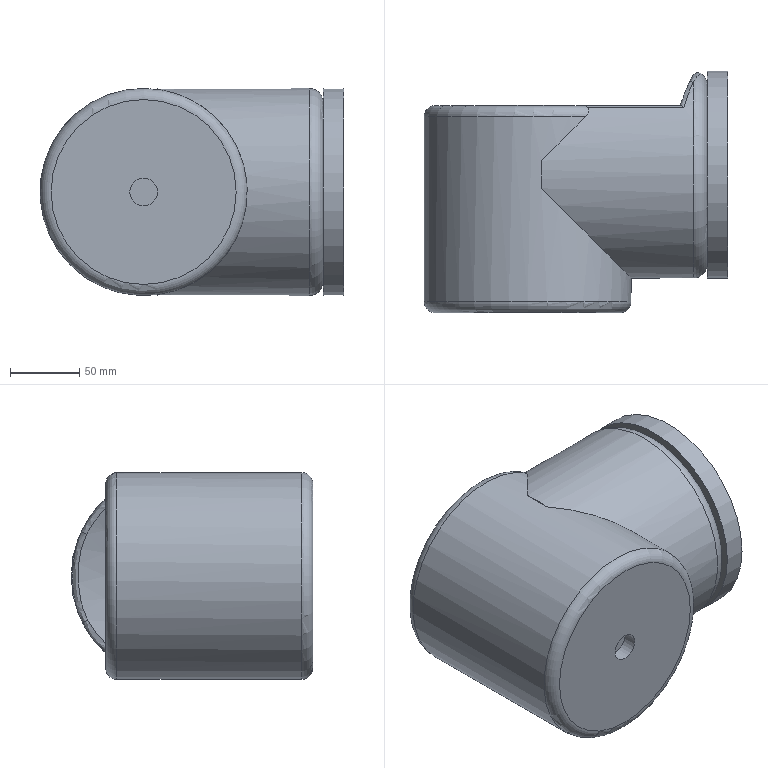Component | NX | 6_WRIST | 2 solids | 26 faces | box 220 x 175 x 150 mm | volume 3966600 mm3 | cylinder 10 | plane 10 | torus 3 | spline 3 | commonest cylinder face diameters 150 x4 20 x3 10 x2 300 x1
STEP:
#1=CARTESIAN_POINT('',(0.,0.,0.));
#2=DIRECTION('',(0.,0.,1.));
#3=DIRECTION('',(1.,0.,0.));
#4=AXIS2_PLACEMENT_3D('',#1,#2,#3);
#5=(LENGTH_UNIT()NAMED_UNIT(*)SI_UNIT(.MILLI.,.METRE.));
#6=UNCERTAINTY_MEASURE_WITH_UNIT(LENGTH_MEASURE(0.0508),#5,'','');
#7=(NAMED_UNIT(*)PLANE_ANGLE_UNIT()SI_UNIT($,.RADIAN.));
#8=PLANE_ANGLE_MEASURE_WITH_UNIT(PLANE_ANGLE_MEASURE(0.01745),#7);
#9=DIMENSIONAL_EXPONENTS(0.,0.,0.,0.,0.,0.,0.);
#10=(CONVERSION_BASED_UNIT('',#8)NAMED_UNIT(#9)PLANE_ANGLE_UNIT());
#11=(NAMED_UNIT(*)SI_UNIT($,.STERADIAN.)SOLID_ANGLE_UNIT());
#12=(GEOMETRIC_REPRESENTATION_CONTEXT(3)GLOBAL_UNCERTAINTY_ASSIGNED_CONTEXT((#6))GLOBAL_UNIT_ASSIGNED_CONTEXT((#5,#10,#11))REPRESENTATION_CONTEXT('',''));
#13=SHAPE_REPRESENTATION('',(#4),#12);
#14=CARTESIAN_POINT('',(0.,0.,-237.5));
#15=DIRECTION('',(0.,0.,1.));
#16=DIRECTION('',(1.,0.,0.));
#17=AXIS2_PLACEMENT_3D('',#14,#15,#16);
#18=CONSTRUCTIVE_GEOMETRY_REPRESENTATION('',(#17),#12);
#19=CONSTRUCTIVE_GEOMETRY_REPRESENTATION_RELATIONSHIP('','',#13,#18);
#20=VALUE_REPRESENTATION_ITEM('',COUNT_MEASURE(0.));
#21=REPRESENTATION('',(#20),#12);
#22=VALUE_REPRESENTATION_ITEM('',COUNT_MEASURE(0.));
#23=REPRESENTATION('',(#22),#12);
#24=CARTESIAN_POINT('',(1171.262,-87.,1644.589));
#25=VERTEX_POINT('',#24);
#26=CARTESIAN_POINT('',(1171.262,-87.,1569.589));
#27=DIRECTION('',(0.,1.,0.));
#28=DIRECTION('',(0.,0.,1.));
#29=AXIS2_PLACEMENT_3D('',#26,#27,#28);
#30=CIRCLE('',#29,75.);
#31=EDGE_CURVE('',#25,#25,#30,.T.);
#32=ORIENTED_EDGE('',*,*,#31,.T.);
#33=EDGE_LOOP('',(#32));
#34=FACE_BOUND('',#33,.T.);
#35=CARTESIAN_POINT('',(1181.262,15.,1495.259));
#36=VERTEX_POINT('',#35);
#37=CARTESIAN_POINT('',(1213.262,47.,1507.452));
#38=VERTEX_POINT('',#37);
#39=CARTESIAN_POINT('',(1171.262,5.,1569.589));
#40=DIRECTION('',(0.7071,-0.7071,0.));
#41=DIRECTION('',(0.7071,0.7071,0.));
#42=AXIS2_PLACEMENT_3D('',#39,#40,#41);
#43=ELLIPSE('',#42,106.066,75.);
#44=EDGE_CURVE('',#36,#38,#43,.T.);
#45=ORIENTED_EDGE('',*,*,#44,.F.);
#46=CARTESIAN_POINT('',(1181.262,-5.,1495.259));
#47=VERTEX_POINT('',#46);
#48=CARTESIAN_POINT('',(1181.262,-95.,1495.259));
#49=DIRECTION('',(0.,1.,0.));
#50=VECTOR('',#49,1.);
#51=LINE('',#48,#50);
#52=EDGE_CURVE('',#47,#36,#51,.T.);
#53=ORIENTED_EDGE('',*,*,#52,.F.);
#54=CARTESIAN_POINT('',(1181.262,-5.,1643.92));
#55=VERTEX_POINT('',#54);
#56=CARTESIAN_POINT('',(1171.262,5.,1569.589));
#57=DIRECTION('',(0.7071,0.7071,0.));
#58=DIRECTION('',(-0.7071,0.7071,0.));
#59=AXIS2_PLACEMENT_3D('',#56,#57,#58);
#60=ELLIPSE('',#59,106.066,75.);
#61=EDGE_CURVE('',#55,#47,#60,.T.);
#62=ORIENTED_EDGE('',*,*,#61,.F.);
#63=CARTESIAN_POINT('',(1181.262,15.,1643.92));
#64=VERTEX_POINT('',#63);
#65=CARTESIAN_POINT('',(1181.262,-95.,1643.92));
#66=DIRECTION('',(0.,-1.,0.));
#67=VECTOR('',#66,1.);
#68=LINE('',#65,#67);
#69=EDGE_CURVE('',#64,#55,#68,.T.);
#70=ORIENTED_EDGE('',*,*,#69,.F.);
#71=CARTESIAN_POINT('',(1213.262,47.,1631.726));
#72=VERTEX_POINT('',#71);
#73=CARTESIAN_POINT('',(1171.262,5.,1569.589));
#74=DIRECTION('',(0.7071,-0.7071,0.));
#75=DIRECTION('',(0.7071,0.7071,0.));
#76=AXIS2_PLACEMENT_3D('',#73,#74,#75);
#77=ELLIPSE('',#76,106.066,75.);
#78=EDGE_CURVE('',#72,#64,#77,.T.);
#79=ORIENTED_EDGE('',*,*,#78,.F.);
#80=CARTESIAN_POINT('',(1171.262,47.,1569.589));
#81=DIRECTION('',(0.,-1.,0.));
#82=DIRECTION('',(0.,0.,1.));
#83=AXIS2_PLACEMENT_3D('',#80,#81,#82);
#84=CIRCLE('',#83,75.);
#85=EDGE_CURVE('',#72,#38,#84,.T.);
#86=ORIENTED_EDGE('',*,*,#85,.T.);
#87=EDGE_LOOP('',(#45,#53,#62,#70,#79,#86));
#88=FACE_BOUND('',#87,.T.);
#89=CARTESIAN_POINT('',(1171.262,-95.,1569.589));
#90=DIRECTION('',(0.,1.,0.));
#91=DIRECTION('',(0.,0.,-1.));
#92=AXIS2_PLACEMENT_3D('',#89,#90,#91);
#93=CYLINDRICAL_SURFACE('',#92,75.);
#94=ADVANCED_FACE('',(#34,#88),#93,.T.);
#95=CARTESIAN_POINT('',(1214.726,53.214,1512.14));
#96=VERTEX_POINT('',#95);
#97=CARTESIAN_POINT('',(1211.436,55.,1515.97));
#98=VERTEX_POINT('',#97);
#99=CARTESIAN_POINT('',(1214.726,53.214,1512.14));
#100=CARTESIAN_POINT('',(1213.654,54.361,1513.102));
#101=CARTESIAN_POINT('',(1212.548,55.,1514.535));
#102=CARTESIAN_POINT('',(1211.436,55.,1515.97));
#103=B_SPLINE_CURVE_WITH_KNOTS('',3,(#99,#100,#101,#102),.UNSPECIFIED.,.F.,.F.,(4,4),(0.,1.),.UNSPECIFIED.);
#104=EDGE_CURVE('',#96,#98,#103,.T.);
#105=ORIENTED_EDGE('',*,*,#104,.F.);
#106=CARTESIAN_POINT('',(1214.726,53.214,1512.14));
#107=CARTESIAN_POINT('',(1215.561,52.321,1511.39));
#108=CARTESIAN_POINT('',(1215.653,51.105,1510.418));
#109=CARTESIAN_POINT('',(1214.918,48.916,1508.776));
#110=CARTESIAN_POINT('',(1214.17,47.908,1508.066));
#111=CARTESIAN_POINT('',(1213.262,47.,1507.452));
#112=B_SPLINE_CURVE_WITH_KNOTS('',3,(#106,#107,#108,#109,#110,#111),.UNSPECIFIED.,.F.,.F.,(4,2,4),(0.,0.5,1.),.UNSPECIFIED.);
#113=EDGE_CURVE('',#96,#38,#112,.T.);
#114=ORIENTED_EDGE('',*,*,#113,.T.);
#115=ORIENTED_EDGE('',*,*,#85,.F.);
#116=CARTESIAN_POINT('',(1214.726,53.214,1627.038));
#117=VERTEX_POINT('',#116);
#118=CARTESIAN_POINT('',(1213.262,47.,1631.726));
#119=CARTESIAN_POINT('',(1214.171,47.909,1631.112));
#120=CARTESIAN_POINT('',(1214.92,48.919,1630.4));
#121=CARTESIAN_POINT('',(1215.654,51.11,1628.756));
#122=CARTESIAN_POINT('',(1215.562,52.32,1627.789));
#123=CARTESIAN_POINT('',(1214.726,53.214,1627.038));
#124=B_SPLINE_CURVE_WITH_KNOTS('',3,(#118,#119,#120,#121,#122,#123),.UNSPECIFIED.,.F.,.F.,(4,2,4),(0.,0.5,1.),.UNSPECIFIED.);
#125=EDGE_CURVE('',#72,#117,#124,.T.);
#126=ORIENTED_EDGE('',*,*,#125,.T.);
#127=CARTESIAN_POINT('',(1211.436,55.,1623.208));
#128=VERTEX_POINT('',#127);
#129=CARTESIAN_POINT('',(1211.436,55.,1623.208));
#130=CARTESIAN_POINT('',(1212.549,55.,1624.644));
#131=CARTESIAN_POINT('',(1213.654,54.361,1626.076));
#132=CARTESIAN_POINT('',(1214.726,53.214,1627.038));
#133=B_SPLINE_CURVE_WITH_KNOTS('',3,(#129,#130,#131,#132),.UNSPECIFIED.,.F.,.F.,(4,4),(0.,1.),.UNSPECIFIED.);
#134=EDGE_CURVE('',#128,#117,#133,.T.);
#135=ORIENTED_EDGE('',*,*,#134,.F.);
#136=CARTESIAN_POINT('',(1171.262,55.,1569.589));
#137=DIRECTION('',(0.,1.,0.));
#138=DIRECTION('',(0.,0.,1.));
#139=AXIS2_PLACEMENT_3D('',#136,#137,#138);
#140=CIRCLE('',#139,67.);
#141=EDGE_CURVE('',#98,#128,#140,.T.);
#142=ORIENTED_EDGE('',*,*,#141,.F.);
#143=EDGE_LOOP('',(#105,#114,#115,#126,#135,#142));
#144=FACE_OUTER_BOUND('',#143,.T.);
#145=CARTESIAN_POINT('',(1171.262,47.,1569.589));
#146=DIRECTION('',(0.,-1.,0.));
#147=DIRECTION('',(0.,0.,1.));
#148=AXIS2_PLACEMENT_3D('',#145,#146,#147);
#149=TOROIDAL_SURFACE('',#148,67.,8.);
#150=ADVANCED_FACE('',(#144),#149,.T.);
#151=CARTESIAN_POINT('',(1171.262,-95.,1636.589));
#152=VERTEX_POINT('',#151);
#153=CARTESIAN_POINT('',(1171.262,-95.,1569.589));
#154=DIRECTION('',(0.,-1.,0.));
#155=DIRECTION('',(0.,0.,1.));
#156=AXIS2_PLACEMENT_3D('',#153,#154,#155);
#157=CIRCLE('',#156,67.);
#158=EDGE_CURVE('',#152,#152,#157,.T.);
#159=ORIENTED_EDGE('',*,*,#158,.T.);
#160=EDGE_LOOP('',(#159));
#161=FACE_BOUND('',#160,.T.);
#162=CARTESIAN_POINT('',(1161.262,-95.,1569.589));
#163=VERTEX_POINT('',#162);
#164=CARTESIAN_POINT('',(1171.262,-95.,1569.589));
#165=DIRECTION('',(0.,1.,0.));
#166=DIRECTION('',(-1.,0.,0.));
#167=AXIS2_PLACEMENT_3D('',#164,#165,#166);
#168=CIRCLE('',#167,10.);
#169=EDGE_CURVE('',#163,#163,#168,.T.);
#170=ORIENTED_EDGE('',*,*,#169,.T.);
#171=EDGE_LOOP('',(#170));
#172=FACE_BOUND('',#171,.T.);
#173=CARTESIAN_POINT('',(1171.262,-95.,1569.589));
#174=DIRECTION('',(0.,-1.,0.));
#175=DIRECTION('',(0.,0.,1.));
#176=AXIS2_PLACEMENT_3D('',#173,#174,#175);
#177=PLANE('',#176);
#178=ADVANCED_FACE('',(#161,#172),#177,.T.);
#179=ORIENTED_EDGE('',*,*,#141,.T.);
#180=CARTESIAN_POINT('',(1281.893,55.,1623.208));
#181=VERTEX_POINT('',#180);
#182=CARTESIAN_POINT('',(1279.425,55.,1623.208));
#183=DIRECTION('',(1.,0.,0.));
#184=VECTOR('',#183,1.);
#185=LINE('',#182,#184);
#186=EDGE_CURVE('',#128,#181,#185,.T.);
#187=ORIENTED_EDGE('',*,*,#186,.T.);
#188=CARTESIAN_POINT('',(1282.026,55.,1618.665));
#189=VERTEX_POINT('',#188);
#190=CARTESIAN_POINT('',(1281.893,55.,1623.208));
#191=CARTESIAN_POINT('',(1281.349,55.,1621.739));
#192=CARTESIAN_POINT('',(1281.508,55.,1620.133));
#193=CARTESIAN_POINT('',(1282.026,55.,1618.665));
#194=B_SPLINE_CURVE_WITH_KNOTS('',3,(#190,#191,#192,#193),.UNSPECIFIED.,.F.,.F.,(4,4),(0.,1.),.UNSPECIFIED.);
#195=EDGE_CURVE('',#181,#189,#194,.T.);
#196=ORIENTED_EDGE('',*,*,#195,.T.);
#197=CARTESIAN_POINT('',(1282.635,55.,1520.467));
#198=VERTEX_POINT('',#197);
#199=CARTESIAN_POINT('',(1140.597,55.,1568.688));
#200=DIRECTION('',(0.,1.,0.));
#201=DIRECTION('',(1.,0.,0.));
#202=AXIS2_PLACEMENT_3D('',#199,#200,#201);
#203=CIRCLE('',#202,150.);
#204=EDGE_CURVE('',#189,#198,#203,.T.);
#205=ORIENTED_EDGE('',*,*,#204,.T.);
#206=CARTESIAN_POINT('',(1282.546,55.,1515.97));
#207=VERTEX_POINT('',#206);
#208=CARTESIAN_POINT('',(1282.635,55.,1520.467));
#209=CARTESIAN_POINT('',(1282.14,55.,1519.009));
#210=CARTESIAN_POINT('',(1282.002,55.,1517.42));
#211=CARTESIAN_POINT('',(1282.546,55.,1515.97));
#212=B_SPLINE_CURVE_WITH_KNOTS('',3,(#208,#209,#210,#211),.UNSPECIFIED.,.F.,.F.,(4,4),(0.,1.),.UNSPECIFIED.);
#213=EDGE_CURVE('',#198,#207,#212,.T.);
#214=ORIENTED_EDGE('',*,*,#213,.T.);
#215=CARTESIAN_POINT('',(1181.262,55.,1515.97));
#216=DIRECTION('',(-1.,0.,0.));
#217=VECTOR('',#216,1.);
#218=LINE('',#215,#217);
#219=EDGE_CURVE('',#207,#98,#218,.T.);
#220=ORIENTED_EDGE('',*,*,#219,.T.);
#221=EDGE_LOOP('',(#179,#187,#196,#205,#214,#220));
#222=FACE_BOUND('',#221,.T.);
#223=CARTESIAN_POINT('',(1171.262,55.,1579.589));
#224=VERTEX_POINT('',#223);
#225=CARTESIAN_POINT('',(1171.262,55.,1569.589));
#226=DIRECTION('',(0.,-1.,0.));
#227=DIRECTION('',(0.,0.,1.));
#228=AXIS2_PLACEMENT_3D('',#225,#226,#227);
#229=CIRCLE('',#228,10.);
#230=EDGE_CURVE('',#224,#224,#229,.T.);
#231=ORIENTED_EDGE('',*,*,#230,.T.);
#232=EDGE_LOOP('',(#231));
#233=FACE_BOUND('',#232,.T.);
#234=CARTESIAN_POINT('',(1171.262,55.,1569.589));
#235=DIRECTION('',(0.,-1.,0.));
#236=DIRECTION('',(0.,0.,1.));
#237=AXIS2_PLACEMENT_3D('',#234,#235,#236);
#238=PLANE('',#237);
#239=ADVANCED_FACE('',(#222,#233),#238,.F.);
#240=ORIENTED_EDGE('',*,*,#230,.F.);
#241=EDGE_LOOP('',(#240));
#242=FACE_BOUND('',#241,.T.);
#243=CARTESIAN_POINT('',(1171.262,45.,1579.589));
#244=VERTEX_POINT('',#243);
#245=CARTESIAN_POINT('',(1171.262,45.,1569.589));
#246=DIRECTION('',(0.,-1.,0.));
#247=DIRECTION('',(0.,0.,1.));
#248=AXIS2_PLACEMENT_3D('',#245,#246,#247);
#249=CIRCLE('',#248,10.);
#250=EDGE_CURVE('',#244,#244,#249,.T.);
#251=ORIENTED_EDGE('',*,*,#250,.T.);
#252=EDGE_LOOP('',(#251));
#253=FACE_BOUND('',#252,.T.);
#254=CARTESIAN_POINT('',(1171.262,55.,1569.589));
#255=DIRECTION('',(0.,-1.,0.));
#256=DIRECTION('',(0.,0.,1.));
#257=AXIS2_PLACEMENT_3D('',#254,#255,#256);
#258=CYLINDRICAL_SURFACE('',#257,10.);
#259=ADVANCED_FACE('',(#242,#253),#258,.F.);
#260=ORIENTED_EDGE('',*,*,#250,.F.);
#261=EDGE_LOOP('',(#260));
#262=FACE_OUTER_BOUND('',#261,.T.);
#263=CARTESIAN_POINT('',(1171.262,45.,1569.589));
#264=DIRECTION('',(0.,-1.,0.));
#265=DIRECTION('',(0.,0.,1.));
#266=AXIS2_PLACEMENT_3D('',#263,#264,#265);
#267=PLANE('',#266);
#268=ADVANCED_FACE('',(#262),#267,.F.);
#269=ORIENTED_EDGE('',*,*,#169,.F.);
#270=EDGE_LOOP('',(#269));
#271=FACE_BOUND('',#270,.T.);
#272=CARTESIAN_POINT('',(1161.262,-85.,1569.589));
#273=VERTEX_POINT('',#272);
#274=CARTESIAN_POINT('',(1171.262,-85.,1569.589));
#275=DIRECTION('',(0.,1.,0.));
#276=DIRECTION('',(-1.,0.,0.));
#277=AXIS2_PLACEMENT_3D('',#274,#275,#276);
#278=CIRCLE('',#277,10.);
#279=EDGE_CURVE('',#273,#273,#278,.T.);
#280=ORIENTED_EDGE('',*,*,#279,.T.);
#281=EDGE_LOOP('',(#280));
#282=FACE_BOUND('',#281,.T.);
#283=CARTESIAN_POINT('',(1171.262,-95.,1569.589));
#284=DIRECTION('',(0.,1.,0.));
#285=DIRECTION('',(0.,0.,-1.));
#286=AXIS2_PLACEMENT_3D('',#283,#284,#285);
#287=CYLINDRICAL_SURFACE('',#286,10.);
#288=ADVANCED_FACE('',(#271,#282),#287,.F.);
#289=ORIENTED_EDGE('',*,*,#279,.F.);
#290=EDGE_LOOP('',(#289));
#291=FACE_OUTER_BOUND('',#290,.T.);
#292=CARTESIAN_POINT('',(1171.262,-85.,1569.589));
#293=DIRECTION('',(0.,1.,0.));
#294=DIRECTION('',(0.,0.,-1.));
#295=AXIS2_PLACEMENT_3D('',#292,#293,#294);
#296=PLANE('',#295);
#297=ADVANCED_FACE('',(#291),#296,.F.);
#298=ORIENTED_EDGE('',*,*,#31,.F.);
#299=EDGE_LOOP('',(#298));
#300=FACE_BOUND('',#299,.T.);
#301=ORIENTED_EDGE('',*,*,#158,.F.);
#302=EDGE_LOOP('',(#301));
#303=FACE_BOUND('',#302,.T.);
#304=CARTESIAN_POINT('',(1171.262,-87.,1569.589));
#305=DIRECTION('',(0.,-1.,0.));
#306=DIRECTION('',(0.,0.,1.));
#307=AXIS2_PLACEMENT_3D('',#304,#305,#306);
#308=TOROIDAL_SURFACE('',#307,67.,8.);
#309=ADVANCED_FACE('',(#300,#303),#308,.T.);
#310=CARTESIAN_POINT('',(1181.262,5.,1569.589));
#311=DIRECTION('',(1.,0.,0.));
#312=DIRECTION('',(0.,-1.,0.));
#313=AXIS2_PLACEMENT_3D('',#310,#311,#312);
#314=CIRCLE('',#313,75.);
#315=EDGE_CURVE('',#47,#36,#314,.T.);
#316=ORIENTED_EDGE('',*,*,#315,.F.);
#317=ORIENTED_EDGE('',*,*,#52,.T.);
#318=EDGE_LOOP('',(#316,#317));
#319=FACE_OUTER_BOUND('',#318,.T.);
#320=CARTESIAN_POINT('',(1181.262,5.,1569.589));
#321=DIRECTION('',(1.,0.,0.));
#322=DIRECTION('',(0.,0.,1.));
#323=AXIS2_PLACEMENT_3D('',#320,#321,#322);
#324=PLANE('',#323);
#325=ADVANCED_FACE('',(#319),#324,.F.);
#326=CARTESIAN_POINT('',(1181.262,5.,1569.589));
#327=DIRECTION('',(1.,0.,0.));
#328=DIRECTION('',(0.,-1.,0.));
#329=AXIS2_PLACEMENT_3D('',#326,#327,#328);
#330=CIRCLE('',#329,75.);
#331=EDGE_CURVE('',#64,#55,#330,.T.);
#332=ORIENTED_EDGE('',*,*,#331,.F.);
#333=ORIENTED_EDGE('',*,*,#69,.T.);
#334=EDGE_LOOP('',(#332,#333));
#335=FACE_OUTER_BOUND('',#334,.T.);
#336=CARTESIAN_POINT('',(1181.262,5.,1569.589));
#337=DIRECTION('',(1.,0.,0.));
#338=DIRECTION('',(0.,0.,1.));
#339=AXIS2_PLACEMENT_3D('',#336,#337,#338);
#340=PLANE('',#339);
#341=ADVANCED_FACE('',(#335),#340,.F.);
#342=ORIENTED_EDGE('',*,*,#331,.T.);
#343=ORIENTED_EDGE('',*,*,#61,.T.);
#344=ORIENTED_EDGE('',*,*,#315,.T.);
#345=ORIENTED_EDGE('',*,*,#44,.T.);
#346=ORIENTED_EDGE('',*,*,#113,.F.);
#347=CARTESIAN_POINT('',(1285.011,53.214,1512.14));
#348=VERTEX_POINT('',#347);
#349=CARTESIAN_POINT('',(1301.262,53.214,1512.14));
#350=DIRECTION('',(1.,0.,0.));
#351=VECTOR('',#350,1.);
#352=LINE('',#349,#351);
#353=EDGE_CURVE('',#96,#348,#352,.T.);
#354=ORIENTED_EDGE('',*,*,#353,.T.);
#355=CARTESIAN_POINT('',(1291.262,71.53,1534.965));
#356=VERTEX_POINT('',#355);
#357=CARTESIAN_POINT('',(1285.011,53.214,1512.14));
#358=CARTESIAN_POINT('',(1286.122,56.989,1515.309));
#359=CARTESIAN_POINT('',(1287.243,60.411,1518.807));
#360=CARTESIAN_POINT('',(1289.385,66.571,1526.482));
#361=CARTESIAN_POINT('',(1290.392,69.269,1530.621));
#362=CARTESIAN_POINT('',(1291.262,71.53,1534.965));
#363=B_SPLINE_CURVE_WITH_KNOTS('',3,(#357,#358,#359,#360,#361,#362),.UNSPECIFIED.,.F.,.F.,(4,2,4),(0.,0.5,1.),.UNSPECIFIED.);
#364=EDGE_CURVE('',#348,#356,#363,.T.);
#365=ORIENTED_EDGE('',*,*,#364,.T.);
#366=CARTESIAN_POINT('',(1291.262,72.487,1602.308));
#367=VERTEX_POINT('',#366);
#368=CARTESIAN_POINT('',(1291.262,5.,1569.589));
#369=DIRECTION('',(-1.,0.,0.));
#370=DIRECTION('',(0.,0.,1.));
#371=AXIS2_PLACEMENT_3D('',#368,#369,#370);
#372=CIRCLE('',#371,75.);
#373=EDGE_CURVE('',#356,#367,#372,.T.);
#374=ORIENTED_EDGE('',*,*,#373,.T.);
#375=CARTESIAN_POINT('',(1284.331,53.214,1627.038));
#376=VERTEX_POINT('',#375);
#377=CARTESIAN_POINT('',(1291.262,72.487,1602.308));
#378=CARTESIAN_POINT('',(1290.3,70.158,1607.111));
#379=CARTESIAN_POINT('',(1289.194,67.373,1611.566));
#380=CARTESIAN_POINT('',(1286.832,60.936,1619.824));
#381=CARTESIAN_POINT('',(1285.567,57.259,1623.644));
#382=CARTESIAN_POINT('',(1284.331,53.214,1627.038));
#383=B_SPLINE_CURVE_WITH_KNOTS('',3,(#377,#378,#379,#380,#381,#382),.UNSPECIFIED.,.F.,.F.,(4,2,4),(0.,0.5,1.),.UNSPECIFIED.);
#384=EDGE_CURVE('',#367,#376,#383,.T.);
#385=ORIENTED_EDGE('',*,*,#384,.T.);
#386=CARTESIAN_POINT('',(1301.262,53.214,1627.038));
#387=DIRECTION('',(-1.,0.,0.));
#388=VECTOR('',#387,1.);
#389=LINE('',#386,#388);
#390=EDGE_CURVE('',#376,#117,#389,.T.);
#391=ORIENTED_EDGE('',*,*,#390,.T.);
#392=ORIENTED_EDGE('',*,*,#125,.F.);
#393=ORIENTED_EDGE('',*,*,#78,.T.);
#394=EDGE_LOOP('',(#342,#343,#344,#345,#346,#354,#365,#374,#385,#391,#392,#393));
#395=FACE_OUTER_BOUND('',#394,.T.);
#396=CARTESIAN_POINT('',(1301.262,5.,1569.589));
#397=DIRECTION('',(-1.,0.,0.));
#398=DIRECTION('',(0.,0.,-1.));
#399=AXIS2_PLACEMENT_3D('',#396,#397,#398);
#400=CYLINDRICAL_SURFACE('',#399,75.);
#401=ADVANCED_FACE('',(#395),#400,.T.);
#402=CARTESIAN_POINT('',(1301.262,5.,1634.589));
#403=VERTEX_POINT('',#402);
#404=CARTESIAN_POINT('',(1301.262,5.,1569.589));
#405=DIRECTION('',(1.,0.,0.));
#406=DIRECTION('',(0.,0.,1.));
#407=AXIS2_PLACEMENT_3D('',#404,#405,#406);
#408=CIRCLE('',#407,65.);
#409=EDGE_CURVE('',#403,#403,#408,.T.);
#410=ORIENTED_EDGE('',*,*,#409,.T.);
#411=EDGE_LOOP('',(#410));
#412=FACE_OUTER_BOUND('',#411,.T.);
#413=CARTESIAN_POINT('',(1301.262,5.,1569.589));
#414=DIRECTION('',(1.,0.,0.));
#415=DIRECTION('',(0.,0.,1.));
#416=AXIS2_PLACEMENT_3D('',#413,#414,#415);
#417=PLANE('',#416);
#418=ADVANCED_FACE('',(#412),#417,.T.);
#419=ORIENTED_EDGE('',*,*,#204,.F.);
#420=CARTESIAN_POINT('',(1287.348,68.887,1599.735));
#421=VERTEX_POINT('',#420);
#422=CARTESIAN_POINT('',(1282.026,55.,1618.665));
#423=CARTESIAN_POINT('',(1283.963,60.672,1613.185));
#424=CARTESIAN_POINT('',(1285.837,65.331,1606.881));
#425=CARTESIAN_POINT('',(1287.348,68.887,1599.735));
#426=B_SPLINE_CURVE_WITH_KNOTS('',3,(#422,#423,#424,#425),.UNSPECIFIED.,.F.,.F.,(4,4),(0.,1.),.UNSPECIFIED.);
#427=EDGE_CURVE('',#189,#421,#426,.T.);
#428=ORIENTED_EDGE('',*,*,#427,.T.);
#429=CARTESIAN_POINT('',(1287.348,67.981,1537.64));
#430=VERTEX_POINT('',#429);
#431=CARTESIAN_POINT('',(1287.348,68.887,1599.735));
#432=CARTESIAN_POINT('',(1288.358,71.263,1594.963));
#433=CARTESIAN_POINT('',(1289.198,72.828,1589.8));
#434=CARTESIAN_POINT('',(1290.316,74.71,1579.284));
#435=CARTESIAN_POINT('',(1290.601,75.058,1573.955));
#436=CARTESIAN_POINT('',(1290.593,74.902,1563.184));
#437=CARTESIAN_POINT('',(1290.294,74.39,1557.826));
#438=CARTESIAN_POINT('',(1289.179,72.212,1547.461));
#439=CARTESIAN_POINT('',(1288.345,70.499,1542.352));
#440=CARTESIAN_POINT('',(1287.348,67.981,1537.64));
#441=B_SPLINE_CURVE_WITH_KNOTS('',3,(#431,#432,#433,#434,#435,#436,#437,#438,#439,#440),.UNSPECIFIED.,.F.,.F.,(4,2,2,2,4),(0.,0.25,0.5,0.75,1.),.UNSPECIFIED.);
#442=EDGE_CURVE('',#421,#430,#441,.T.);
#443=ORIENTED_EDGE('',*,*,#442,.T.);
#444=CARTESIAN_POINT('',(1287.348,67.981,1537.64));
#445=CARTESIAN_POINT('',(1286.009,64.598,1531.307));
#446=CARTESIAN_POINT('',(1284.338,60.194,1525.485));
#447=CARTESIAN_POINT('',(1282.635,55.,1520.467));
#448=B_SPLINE_CURVE_WITH_KNOTS('',3,(#444,#445,#446,#447),.UNSPECIFIED.,.F.,.F.,(4,4),(0.,1.),.UNSPECIFIED.);
#449=EDGE_CURVE('',#430,#198,#448,.T.);
#450=ORIENTED_EDGE('',*,*,#449,.T.);
#451=EDGE_LOOP('',(#419,#428,#443,#450));
#452=FACE_OUTER_BOUND('',#451,.T.);
#453=CARTESIAN_POINT('',(1140.597,85.,1568.688));
#454=DIRECTION('',(0.,-1.,0.));
#455=DIRECTION('',(0.,0.,1.));
#456=AXIS2_PLACEMENT_3D('',#453,#454,#455);
#457=CYLINDRICAL_SURFACE('',#456,150.);
#458=ADVANCED_FACE('',(#452),#457,.F.);
#459=ORIENTED_EDGE('',*,*,#373,.F.);
#460=CARTESIAN_POINT('',(1291.262,71.53,1534.965));
#461=CARTESIAN_POINT('',(1292.934,74.137,1539.976));
#462=CARTESIAN_POINT('',(1294.351,75.8,1545.478));
#463=CARTESIAN_POINT('',(1296.295,77.828,1556.864));
#464=CARTESIAN_POINT('',(1296.818,78.229,1562.754));
#465=CARTESIAN_POINT('',(1296.822,78.383,1574.465));
#466=CARTESIAN_POINT('',(1296.315,78.144,1580.249));
#467=CARTESIAN_POINT('',(1294.387,76.452,1591.643));
#468=CARTESIAN_POINT('',(1292.961,74.955,1597.218));
#469=CARTESIAN_POINT('',(1291.262,72.487,1602.308));
#470=B_SPLINE_CURVE_WITH_KNOTS('',3,(#460,#461,#462,#463,#464,#465,#466,#467,#468,#469),.UNSPECIFIED.,.F.,.F.,(4,2,2,2,4),(0.,0.25,0.5,0.75,1.),.UNSPECIFIED.);
#471=EDGE_CURVE('',#356,#367,#470,.T.);
#472=ORIENTED_EDGE('',*,*,#471,.T.);
#473=EDGE_LOOP('',(#459,#472));
#474=FACE_BOUND('',#473,.T.);
#475=ORIENTED_EDGE('',*,*,#409,.F.);
#476=EDGE_LOOP('',(#475));
#477=FACE_BOUND('',#476,.T.);
#478=CARTESIAN_POINT('',(1291.262,5.,1569.589));
#479=DIRECTION('',(1.,0.,0.));
#480=DIRECTION('',(0.,0.,1.));
#481=AXIS2_PLACEMENT_3D('',#478,#479,#480);
#482=TOROIDAL_SURFACE('',#481,65.,10.);
#483=ADVANCED_FACE('',(#474,#477),#482,.T.);
#484=ORIENTED_EDGE('',*,*,#353,.F.);
#485=ORIENTED_EDGE('',*,*,#104,.T.);
#486=ORIENTED_EDGE('',*,*,#219,.F.);
#487=CARTESIAN_POINT('',(1282.546,55.,1515.97));
#488=CARTESIAN_POINT('',(1283.141,55.,1514.387));
#489=CARTESIAN_POINT('',(1284.095,54.275,1513.03));
#490=CARTESIAN_POINT('',(1285.011,53.214,1512.14));
#491=B_SPLINE_CURVE_WITH_KNOTS('',3,(#487,#488,#489,#490),.UNSPECIFIED.,.F.,.F.,(4,4),(0.,1.),.UNSPECIFIED.);
#492=EDGE_CURVE('',#207,#348,#491,.T.);
#493=ORIENTED_EDGE('',*,*,#492,.T.);
#494=EDGE_LOOP('',(#484,#485,#486,#493));
#495=FACE_OUTER_BOUND('',#494,.T.);
#496=CARTESIAN_POINT('',(1301.262,50.,1515.97));
#497=DIRECTION('',(-1.,0.,0.));
#498=DIRECTION('',(0.,0.,-1.));
#499=AXIS2_PLACEMENT_3D('',#496,#497,#498);
#500=CYLINDRICAL_SURFACE('',#499,5.);
#501=ADVANCED_FACE('',(#495),#500,.T.);
#502=ORIENTED_EDGE('',*,*,#186,.F.);
#503=ORIENTED_EDGE('',*,*,#134,.T.);
#504=ORIENTED_EDGE('',*,*,#390,.F.);
#505=CARTESIAN_POINT('',(1284.331,53.214,1627.038));
#506=CARTESIAN_POINT('',(1283.424,54.275,1626.148));
#507=CARTESIAN_POINT('',(1282.48,55.,1624.79));
#508=CARTESIAN_POINT('',(1281.893,55.,1623.208));
#509=B_SPLINE_CURVE_WITH_KNOTS('',3,(#505,#506,#507,#508),.UNSPECIFIED.,.F.,.F.,(4,4),(0.,1.),.UNSPECIFIED.);
#510=EDGE_CURVE('',#376,#181,#509,.T.);
#511=ORIENTED_EDGE('',*,*,#510,.T.);
#512=EDGE_LOOP('',(#502,#503,#504,#511));
#513=FACE_OUTER_BOUND('',#512,.T.);
#514=CARTESIAN_POINT('',(1301.262,50.,1623.208));
#515=DIRECTION('',(-1.,0.,0.));
#516=DIRECTION('',(0.,0.,-1.));
#517=AXIS2_PLACEMENT_3D('',#514,#515,#516);
#518=CYLINDRICAL_SURFACE('',#517,5.);
#519=ADVANCED_FACE('',(#513),#518,.T.);
#520=ORIENTED_EDGE('',*,*,#213,.F.);
#521=ORIENTED_EDGE('',*,*,#449,.F.);
#522=CARTESIAN_POINT('',(1291.262,67.981,1536.812));
#523=DIRECTION('',(0.1845,0.4537,0.8718));
#524=DIRECTION('',(0.,0.8871,-0.4617));
#525=AXIS2_PLACEMENT_3D('',#522,#523,#524);
#526=CIRCLE('',#525,4.);
#527=EDGE_CURVE('',#356,#430,#526,.T.);
#528=ORIENTED_EDGE('',*,*,#527,.F.);
#529=ORIENTED_EDGE('',*,*,#364,.F.);
#530=ORIENTED_EDGE('',*,*,#492,.F.);
#531=EDGE_LOOP('',(#520,#521,#528,#529,#530));
#532=FACE_OUTER_BOUND('',#531,.T.);
#533=CARTESIAN_POINT('',(1281.222,50.515,1516.489));
#534=CARTESIAN_POINT('',(1279.855,54.014,1512.808));
#535=CARTESIAN_POINT('',(1284.972,53.079,1512.027));
#536=CARTESIAN_POINT('',(1282.301,54.09,1519.398));
#537=CARTESIAN_POINT('',(1281.105,57.649,1515.946));
#538=CARTESIAN_POINT('',(1286.08,56.855,1515.181));
#539=CARTESIAN_POINT('',(1283.397,57.347,1522.623));
#540=CARTESIAN_POINT('',(1282.384,61.015,1519.456));
#541=CARTESIAN_POINT('',(1287.205,60.296,1518.679));
#542=CARTESIAN_POINT('',(1285.5,63.234,1529.74));
#543=CARTESIAN_POINT('',(1284.81,67.035,1527.155));
#544=CARTESIAN_POINT('',(1289.364,66.514,1526.398));
#545=CARTESIAN_POINT('',(1286.497,65.832,1533.617));
#546=CARTESIAN_POINT('',(1285.956,69.697,1531.327));
#547=CARTESIAN_POINT('',(1290.388,69.259,1530.602));
#548=CARTESIAN_POINT('',(1287.348,67.981,1537.64));
#549=CARTESIAN_POINT('',(1286.935,71.904,1535.686));
#550=CARTESIAN_POINT('',(1291.262,71.53,1534.965));
#551=(BOUNDED_SURFACE()B_SPLINE_SURFACE(3,2,((#533,#534,#535),(#536,#537,#538),(#539,#540,#541),(#542,#543,#544),(#545,#546,#547),(#548,#549,#550)),.UNSPECIFIED.,.F.,.F.,.F.)B_SPLINE_SURFACE_WITH_KNOTS((4,2,4),(3,3),(0.,0.5,1.),(0.,1.),.UNSPECIFIED.)GEOMETRIC_REPRESENTATION_ITEM()RATIONAL_B_SPLINE_SURFACE(((1.,0.6054,1.),(1.,0.6176,1.),(1.,0.6297,1.),(1.,0.6527,1.),(1.,0.6634,1.),(1.,0.6725,1.)))REPRESENTATION_ITEM('')SURFACE());
#552=ADVANCED_FACE('',(#532),#551,.T.);
#553=ORIENTED_EDGE('',*,*,#527,.T.);
#554=ORIENTED_EDGE('',*,*,#442,.F.);
#555=CARTESIAN_POINT('',(1291.262,68.887,1600.563));
#556=DIRECTION('',(-0.187,-0.4286,0.8839));
#557=DIRECTION('',(0.,0.8998,0.4363));
#558=AXIS2_PLACEMENT_3D('',#555,#556,#557);
#559=CIRCLE('',#558,4.);
#560=EDGE_CURVE('',#367,#421,#559,.T.);
#561=ORIENTED_EDGE('',*,*,#560,.F.);
#562=ORIENTED_EDGE('',*,*,#471,.F.);
#563=EDGE_LOOP('',(#553,#554,#561,#562));
#564=FACE_OUTER_BOUND('',#563,.T.);
#565=CARTESIAN_POINT('',(1291.262,72.487,1602.308));
#566=CARTESIAN_POINT('',(1286.96,72.844,1601.571));
#567=CARTESIAN_POINT('',(1287.348,68.887,1599.735));
#568=CARTESIAN_POINT('',(1292.987,74.992,1597.14));
#569=CARTESIAN_POINT('',(1288.148,76.227,1596.277));
#570=CARTESIAN_POINT('',(1288.356,71.257,1594.975));
#571=CARTESIAN_POINT('',(1294.43,76.496,1591.455));
#572=CARTESIAN_POINT('',(1289.052,78.487,1590.838));
#573=CARTESIAN_POINT('',(1289.2,72.832,1589.784));
#574=CARTESIAN_POINT('',(1296.34,78.16,1580.038));
#575=CARTESIAN_POINT('',(1290.326,81.792,1579.568));
#576=CARTESIAN_POINT('',(1290.316,74.711,1579.275));
#577=CARTESIAN_POINT('',(1296.827,78.385,1574.307));
#578=CARTESIAN_POINT('',(1290.605,82.552,1574.26));
#579=CARTESIAN_POINT('',(1290.601,75.058,1573.952));
#580=CARTESIAN_POINT('',(1296.817,78.266,1565.633));
#581=CARTESIAN_POINT('',(1290.593,82.423,1565.577));
#582=CARTESIAN_POINT('',(1290.595,74.942,1565.887));
#583=CARTESIAN_POINT('',(1296.688,78.14,1562.731));
#584=CARTESIAN_POINT('',(1290.508,82.146,1562.739));
#585=CARTESIAN_POINT('',(1290.52,74.79,1563.19));
#586=CARTESIAN_POINT('',(1296.194,77.678,1557.001));
#587=CARTESIAN_POINT('',(1290.173,81.14,1557.039));
#588=CARTESIAN_POINT('',(1290.231,74.244,1557.881));
#589=CARTESIAN_POINT('',(1295.828,77.339,1554.157));
#590=CARTESIAN_POINT('',(1289.934,80.448,1554.267));
#591=CARTESIAN_POINT('',(1290.017,73.849,1555.256));
#592=CARTESIAN_POINT('',(1294.399,75.853,1545.704));
#593=CARTESIAN_POINT('',(1289.009,77.845,1546.258));
#594=CARTESIAN_POINT('',(1289.182,72.219,1547.483));
#595=CARTESIAN_POINT('',(1292.986,74.217,1540.129));
#596=CARTESIAN_POINT('',(1288.122,75.48,1540.958));
#597=CARTESIAN_POINT('',(1288.355,70.523,1542.397));
#598=CARTESIAN_POINT('',(1291.262,71.53,1534.965));
#599=CARTESIAN_POINT('',(1286.935,71.904,1535.686));
#600=CARTESIAN_POINT('',(1287.348,67.981,1537.64));
#601=(BOUNDED_SURFACE()B_SPLINE_SURFACE(3,2,((#565,#566,#567),(#568,#569,#570),(#571,#572,#573),(#574,#575,#576),(#577,#578,#579),(#580,#581,#582),(#583,#584,#585),(#586,#587,#588),(#589,#590,#591),(#592,#593,#594),(#595,#596,#597),(#598,#599,#600)),.UNSPECIFIED.,.F.,.F.,.F.)B_SPLINE_SURFACE_WITH_KNOTS((4,2,2,2,2,4),(3,3),(0.,0.25,0.5,0.625,0.75,1.),(0.,1.),.UNSPECIFIED.)GEOMETRIC_REPRESENTATION_ITEM()RATIONAL_B_SPLINE_SURFACE(((1.,0.6744,1.),(1.,0.6226,1.),(1.,0.5715,1.),(1.,0.4953,1.),(1.,0.4711,1.),(1.,0.4713,1.),(1.,0.4773,1.),(1.,0.4991,1.),(1.,0.5148,1.),(1.,0.5711,1.),(1.,0.6209,1.),(1.,0.6725,1.)))REPRESENTATION_ITEM('')SURFACE());
#602=ADVANCED_FACE('',(#564),#601,.T.);
#603=ORIENTED_EDGE('',*,*,#510,.F.);
#604=ORIENTED_EDGE('',*,*,#384,.F.);
#605=ORIENTED_EDGE('',*,*,#560,.T.);
#606=ORIENTED_EDGE('',*,*,#427,.F.);
#607=ORIENTED_EDGE('',*,*,#195,.F.);
#608=EDGE_LOOP('',(#603,#604,#605,#606,#607));
#609=FACE_OUTER_BOUND('',#608,.T.);
#610=CARTESIAN_POINT('',(1287.348,68.887,1599.735));
#611=CARTESIAN_POINT('',(1286.96,72.844,1601.571));
#612=CARTESIAN_POINT('',(1291.262,72.487,1602.308));
#613=CARTESIAN_POINT('',(1286.403,66.663,1604.204));
#614=CARTESIAN_POINT('',(1285.877,70.564,1606.412));
#615=CARTESIAN_POINT('',(1290.291,70.137,1607.154));
#616=CARTESIAN_POINT('',(1285.317,64.003,1608.338));
#617=CARTESIAN_POINT('',(1284.633,67.842,1610.855));
#618=CARTESIAN_POINT('',(1289.176,67.328,1611.638));
#619=CARTESIAN_POINT('',(1282.997,57.852,1615.999));
#620=CARTESIAN_POINT('',(1281.964,61.564,1619.137));
#621=CARTESIAN_POINT('',(1286.794,60.83,1619.946));
#622=CARTESIAN_POINT('',(1281.75,54.32,1619.548));
#623=CARTESIAN_POINT('',(1280.512,57.917,1622.998));
#624=CARTESIAN_POINT('',(1285.514,57.099,1623.795));
#625=CARTESIAN_POINT('',(1280.554,50.506,1622.65));
#626=CARTESIAN_POINT('',(1279.131,54.048,1626.342));
#627=CARTESIAN_POINT('',(1284.287,53.07,1627.159));
#628=(BOUNDED_SURFACE()B_SPLINE_SURFACE(3,2,((#610,#611,#612),(#613,#614,#615),(#616,#617,#618),(#619,#620,#621),(#622,#623,#624),(#625,#626,#627)),.UNSPECIFIED.,.F.,.F.,.F.)B_SPLINE_SURFACE_WITH_KNOTS((4,2,4),(3,3),(0.,0.5,1.),(0.,1.),.UNSPECIFIED.)GEOMETRIC_REPRESENTATION_ITEM()RATIONAL_B_SPLINE_SURFACE(((1.,0.6744,1.),(1.,0.6646,1.),(1.,0.6533,1.),(1.,0.6285,1.),(1.,0.6149,1.),(1.,0.6016,1.)))REPRESENTATION_ITEM('')SURFACE());
#629=ADVANCED_FACE('',(#609),#628,.T.);
#630=CLOSED_SHELL('',(#94,#150,#178,#239,#259,#268,#288,#297,#309,#325,#341,#401,#418,#458,#483,#501,#519,#552,#602,#629));
#631=MANIFOLD_SOLID_BREP('',#630);
#632=CARTESIAN_POINT('',(1316.262,-70.,1569.589));
#633=VERTEX_POINT('',#632);
#634=CARTESIAN_POINT('',(1316.262,5.,1569.589));
#635=DIRECTION('',(1.,0.,0.));
#636=DIRECTION('',(0.,-1.,0.));
#637=AXIS2_PLACEMENT_3D('',#634,#635,#636);
#638=CIRCLE('',#637,75.);
#639=EDGE_CURVE('',#633,#633,#638,.T.);
#640=ORIENTED_EDGE('',*,*,#639,.F.);
#641=EDGE_LOOP('',(#640));
#642=FACE_BOUND('',#641,.T.);
#643=CARTESIAN_POINT('',(1301.262,-70.,1569.589));
#644=VERTEX_POINT('',#643);
#645=CARTESIAN_POINT('',(1301.262,5.,1569.589));
#646=DIRECTION('',(1.,0.,0.));
#647=DIRECTION('',(0.,-1.,0.));
#648=AXIS2_PLACEMENT_3D('',#645,#646,#647);
#649=CIRCLE('',#648,75.);
#650=EDGE_CURVE('',#644,#644,#649,.T.);
#651=ORIENTED_EDGE('',*,*,#650,.T.);
#652=EDGE_LOOP('',(#651));
#653=FACE_BOUND('',#652,.T.);
#654=CARTESIAN_POINT('',(1316.262,5.,1569.589));
#655=DIRECTION('',(-1.,0.,0.));
#656=DIRECTION('',(0.,0.,-1.));
#657=AXIS2_PLACEMENT_3D('',#654,#655,#656);
#658=CYLINDRICAL_SURFACE('',#657,75.);
#659=ADVANCED_FACE('',(#642,#653),#658,.T.);
#660=CARTESIAN_POINT('',(1316.262,-5.,1569.589));
#661=VERTEX_POINT('',#660);
#662=CARTESIAN_POINT('',(1316.262,5.,1569.589));
#663=DIRECTION('',(1.,0.,0.));
#664=DIRECTION('',(0.,-1.,0.));
#665=AXIS2_PLACEMENT_3D('',#662,#663,#664);
#666=CIRCLE('',#665,10.);
#667=EDGE_CURVE('',#661,#661,#666,.T.);
#668=ORIENTED_EDGE('',*,*,#667,.F.);
#669=EDGE_LOOP('',(#668));
#670=FACE_BOUND('',#669,.T.);
#671=ORIENTED_EDGE('',*,*,#639,.T.);
#672=EDGE_LOOP('',(#671));
#673=FACE_BOUND('',#672,.T.);
#674=CARTESIAN_POINT('',(1316.262,5.,1569.589));
#675=DIRECTION('',(1.,0.,0.));
#676=DIRECTION('',(0.,0.,1.));
#677=AXIS2_PLACEMENT_3D('',#674,#675,#676);
#678=PLANE('',#677);
#679=ADVANCED_FACE('',(#670,#673),#678,.T.);
#680=ORIENTED_EDGE('',*,*,#650,.F.);
#681=EDGE_LOOP('',(#680));
#682=FACE_OUTER_BOUND('',#681,.T.);
#683=CARTESIAN_POINT('',(1301.262,5.,1569.589));
#684=DIRECTION('',(1.,0.,0.));
#685=DIRECTION('',(0.,0.,1.));
#686=AXIS2_PLACEMENT_3D('',#683,#684,#685);
#687=PLANE('',#686);
#688=ADVANCED_FACE('',(#682),#687,.F.);
#689=CARTESIAN_POINT('',(1306.262,-5.,1569.589));
#690=VERTEX_POINT('',#689);
#691=CARTESIAN_POINT('',(1306.262,5.,1569.589));
#692=DIRECTION('',(1.,0.,0.));
#693=DIRECTION('',(0.,-1.,0.));
#694=AXIS2_PLACEMENT_3D('',#691,#692,#693);
#695=CIRCLE('',#694,10.);
#696=EDGE_CURVE('',#690,#690,#695,.T.);
#697=ORIENTED_EDGE('',*,*,#696,.F.);
#698=EDGE_LOOP('',(#697));
#699=FACE_BOUND('',#698,.T.);
#700=ORIENTED_EDGE('',*,*,#667,.T.);
#701=EDGE_LOOP('',(#700));
#702=FACE_BOUND('',#701,.T.);
#703=CARTESIAN_POINT('',(1306.262,5.,1569.589));
#704=DIRECTION('',(1.,0.,0.));
#705=DIRECTION('',(0.,0.,1.));
#706=AXIS2_PLACEMENT_3D('',#703,#704,#705);
#707=CYLINDRICAL_SURFACE('',#706,10.);
#708=ADVANCED_FACE('',(#699,#702),#707,.F.);
#709=ORIENTED_EDGE('',*,*,#696,.T.);
#710=EDGE_LOOP('',(#709));
#711=FACE_OUTER_BOUND('',#710,.T.);
#712=CARTESIAN_POINT('',(1306.262,5.,1569.589));
#713=DIRECTION('',(1.,0.,0.));
#714=DIRECTION('',(0.,0.,1.));
#715=AXIS2_PLACEMENT_3D('',#712,#713,#714);
#716=PLANE('',#715);
#717=ADVANCED_FACE('',(#711),#716,.T.);
#718=CLOSED_SHELL('',(#659,#679,#688,#708,#717));
#719=MANIFOLD_SOLID_BREP('',#718);
#720=ADVANCED_BREP_SHAPE_REPRESENTATION('',(#631,#719),#12);
#721=SHAPE_REPRESENTATION_RELATIONSHIP('','',#13,#720);
#722=PRESENTATION_LAYER_ASSIGNMENT('','',(#17,#631,#719));
#723=DRAUGHTING_PRE_DEFINED_CURVE_FONT('');
#724=COLOUR_RGB('',0.6,0.4,0.4);
#725=CURVE_STYLE('',#723,POSITIVE_LENGTH_MEASURE(0.13),#724);
#726=PRESENTATION_STYLE_ASSIGNMENT((#725));
#727=STYLED_ITEM('',(#726),#17);
#728=COLOUR_RGB('',1.,0.4,0.);
#729=FILL_AREA_STYLE_COLOUR('',#728);
#730=FILL_AREA_STYLE('',(#729));
#731=SURFACE_STYLE_FILL_AREA(#730);
#732=SURFACE_SIDE_STYLE('',(#731));
#733=SURFACE_STYLE_USAGE(.BOTH.,#732);
#734=PRESENTATION_STYLE_ASSIGNMENT((#733));
#735=STYLED_ITEM('',(#734),#631);
#736=COLOUR_RGB('',0.5961,0.6667,0.6863);
#737=FILL_AREA_STYLE_COLOUR('',#736);
#738=FILL_AREA_STYLE('',(#737));
#739=SURFACE_STYLE_FILL_AREA(#738);
#740=SURFACE_SIDE_STYLE('',(#739));
#741=SURFACE_STYLE_USAGE(.BOTH.,#740);
#742=PRESENTATION_STYLE_ASSIGNMENT((#741));
#743=STYLED_ITEM('',(#742),#719);
#744=MECHANICAL_DESIGN_GEOMETRIC_PRESENTATION_REPRESENTATION('',(#727,#735,#743),#12);